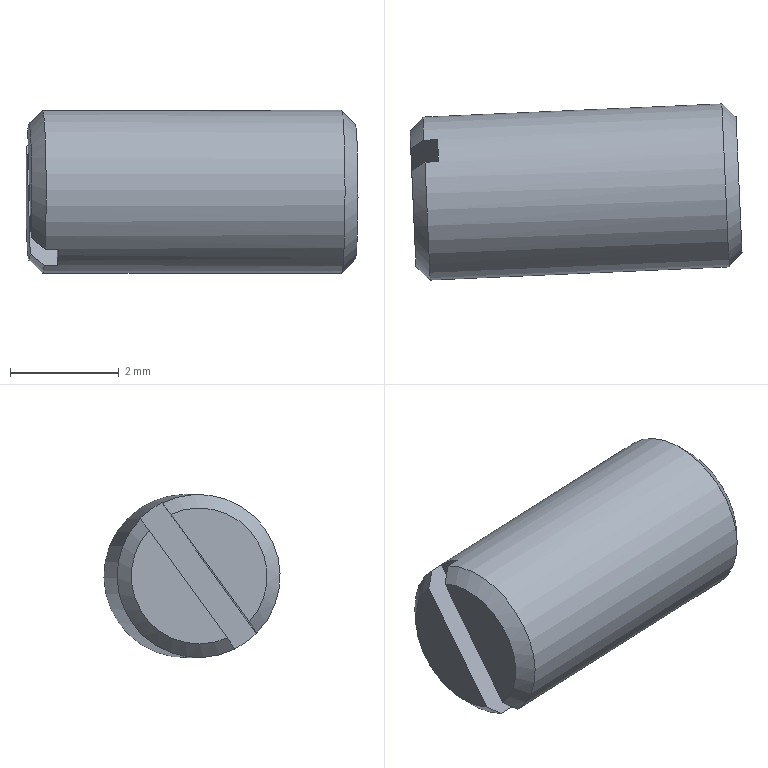Component | NX | SCREW_M3X6 | 1 solid | 10 faces | box 6.1 x 3.24 x 3 mm | volume 41 mm3 | plane 6 | cone 3 | cylinder 1 | commonest cylinder face diameters 3 x1
STEP:
#1=CARTESIAN_POINT('',(0.,0.,0.));
#2=DIRECTION('',(0.,0.,1.));
#3=DIRECTION('',(1.,0.,0.));
#4=AXIS2_PLACEMENT_3D('',#1,#2,#3);
#5=CARTESIAN_POINT('',(-43.719,-0.9021,63.862));
#6=VERTEX_POINT('',#5);
#7=CARTESIAN_POINT('',(-43.782,0.536,65.844));
#8=VERTEX_POINT('',#7);
#9=CARTESIAN_POINT('',(-43.692,-1.51,63.024));
#10=DIRECTION('',(-0.02587,0.5871,0.8091));
#11=VECTOR('',#10,1.);
#12=LINE('',#9,#11);
#13=CARTESIAN_POINT('',(-43.742,-0.3851,65.));
#14=DIRECTION('',(-0.999,-0.04401,0.));
#15=DIRECTION('',(-0.02587,0.5871,0.8091));
#16=AXIS2_PLACEMENT_3D('',#13,#14,#15);
#17=PLANE('',#16);
#18=CARTESIAN_POINT('',(-2.261,0.25));
#19=DIRECTION('',(1.,-0.));
#20=VECTOR('',#19,1.);
#21=LINE('',#18,#20);
#22=(GEOMETRIC_REPRESENTATION_CONTEXT(2)PARAMETRIC_REPRESENTATION_CONTEXT()REPRESENTATION_CONTEXT('',''));
#23=DEFINITIONAL_REPRESENTATION('',(#21),#22);
#24=PCURVE('',#17,#23);
#25=CARTESIAN_POINT('',(-43.192,-1.488,63.024));
#26=DIRECTION('',(0.03561,-0.8083,0.5877));
#27=DIRECTION('',(0.999,0.04401,-0.));
#28=AXIS2_PLACEMENT_3D('',#25,#26,#27);
#29=PLANE('',#28);
#30=CARTESIAN_POINT('',(-0.5,-0.));
#31=DIRECTION('',(0.,1.));
#32=VECTOR('',#31,1.);
#33=LINE('',#30,#32);
#34=(GEOMETRIC_REPRESENTATION_CONTEXT(2)PARAMETRIC_REPRESENTATION_CONTEXT()REPRESENTATION_CONTEXT('',''));
#35=DEFINITIONAL_REPRESENTATION('',(#33),#34);
#36=PCURVE('',#29,#35);
#37=SURFACE_CURVE('',#12,(#24,#36),.PCURVE_S1.);
#38=EDGE_CURVE('',#6,#8,#37,.T.);
#39=ORIENTED_EDGE('',*,*,#38,.T.);
#40=CARTESIAN_POINT('',(-43.742,-0.3851,65.));
#41=DIRECTION('',(-0.999,-0.04401,0.));
#42=DIRECTION('',(-0.02587,0.5871,0.8091));
#43=AXIS2_PLACEMENT_3D('',#40,#41,#42);
#44=CIRCLE('',#43,1.25);
#45=CARTESIAN_POINT('',(0.,0.));
#46=DIRECTION('',(1.,0.));
#47=AXIS2_PLACEMENT_2D('',#45,#46);
#48=CIRCLE('',#47,1.25);
#49=(GEOMETRIC_REPRESENTATION_CONTEXT(2)PARAMETRIC_REPRESENTATION_CONTEXT()REPRESENTATION_CONTEXT('',''));
#50=DEFINITIONAL_REPRESENTATION('',(#48),#49);
#51=PCURVE('',#17,#50);
#52=CARTESIAN_POINT('',(-43.492,-0.3741,65.));
#53=DIRECTION('',(0.999,0.04401,0.));
#54=DIRECTION('',(0.02587,-0.5871,-0.8091));
#55=AXIS2_PLACEMENT_3D('',#52,#53,#54);
#56=CONICAL_SURFACE('',#55,1.5,0.7854);
#57=CARTESIAN_POINT('',(3.142,-0.25));
#58=DIRECTION('',(-1.,0.));
#59=VECTOR('',#58,1.);
#60=LINE('',#57,#59);
#61=(GEOMETRIC_REPRESENTATION_CONTEXT(2)PARAMETRIC_REPRESENTATION_CONTEXT()REPRESENTATION_CONTEXT('',''));
#62=DEFINITIONAL_REPRESENTATION('',(#60),#61);
#63=PCURVE('',#56,#62);
#64=SURFACE_CURVE('',#44,(#51,#63),.PCURVE_S1.);
#65=EDGE_CURVE('',#8,#6,#64,.T.);
#66=ORIENTED_EDGE('',*,*,#65,.T.);
#67=EDGE_LOOP('',(#39,#66));
#68=FACE_BOUND('',#67,.T.);
#69=ADVANCED_FACE('',(#68),#17,.T.);
#70=CARTESIAN_POINT('',(-43.764,0.1318,66.138));
#71=VERTEX_POINT('',#70);
#72=CARTESIAN_POINT('',(-43.701,-1.306,64.156));
#73=VERTEX_POINT('',#72);
#74=CARTESIAN_POINT('',(-43.791,0.7402,66.976));
#75=DIRECTION('',(0.02587,-0.5871,-0.8091));
#76=VECTOR('',#75,1.);
#77=LINE('',#74,#76);
#78=CARTESIAN_POINT('',(-43.742,-0.3851,65.));
#79=DIRECTION('',(-0.999,-0.04401,0.));
#80=DIRECTION('',(-0.02587,0.5871,0.8091));
#81=AXIS2_PLACEMENT_3D('',#78,#79,#80);
#82=PLANE('',#81);
#83=CARTESIAN_POINT('',(2.261,-0.25));
#84=DIRECTION('',(-1.,0.));
#85=VECTOR('',#84,1.);
#86=LINE('',#83,#85);
#87=(GEOMETRIC_REPRESENTATION_CONTEXT(2)PARAMETRIC_REPRESENTATION_CONTEXT()REPRESENTATION_CONTEXT('',''));
#88=DEFINITIONAL_REPRESENTATION('',(#86),#87);
#89=PCURVE('',#82,#88);
#90=CARTESIAN_POINT('',(-43.292,0.7622,66.976));
#91=DIRECTION('',(-0.03561,0.8083,-0.5877));
#92=DIRECTION('',(-0.999,-0.04401,0.));
#93=AXIS2_PLACEMENT_3D('',#90,#91,#92);
#94=PLANE('',#93);
#95=CARTESIAN_POINT('',(0.5,0.));
#96=DIRECTION('',(0.,-1.));
#97=VECTOR('',#96,1.);
#98=LINE('',#95,#97);
#99=(GEOMETRIC_REPRESENTATION_CONTEXT(2)PARAMETRIC_REPRESENTATION_CONTEXT()REPRESENTATION_CONTEXT('',''));
#100=DEFINITIONAL_REPRESENTATION('',(#98),#99);
#101=PCURVE('',#94,#100);
#102=SURFACE_CURVE('',#77,(#89,#101),.PCURVE_S1.);
#103=EDGE_CURVE('',#71,#73,#102,.T.);
#104=ORIENTED_EDGE('',*,*,#103,.T.);
#105=CARTESIAN_POINT('',(-43.742,-0.3851,65.));
#106=DIRECTION('',(-0.999,-0.04401,0.));
#107=DIRECTION('',(-0.02587,0.5871,0.8091));
#108=AXIS2_PLACEMENT_3D('',#105,#106,#107);
#109=CIRCLE('',#108,1.25);
#110=CARTESIAN_POINT('',(0.,0.));
#111=DIRECTION('',(1.,0.));
#112=AXIS2_PLACEMENT_2D('',#110,#111);
#113=CIRCLE('',#112,1.25);
#114=(GEOMETRIC_REPRESENTATION_CONTEXT(2)PARAMETRIC_REPRESENTATION_CONTEXT()REPRESENTATION_CONTEXT('',''));
#115=DEFINITIONAL_REPRESENTATION('',(#113),#114);
#116=PCURVE('',#82,#115);
#117=CARTESIAN_POINT('',(-43.492,-0.3741,65.));
#118=DIRECTION('',(0.999,0.04401,0.));
#119=DIRECTION('',(0.02587,-0.5871,-0.8091));
#120=AXIS2_PLACEMENT_3D('',#117,#118,#119);
#121=CONICAL_SURFACE('',#120,1.5,0.7854);
#122=CARTESIAN_POINT('',(9.425,-0.25));
#123=DIRECTION('',(-1.,0.));
#124=VECTOR('',#123,1.);
#125=LINE('',#122,#124);
#126=(GEOMETRIC_REPRESENTATION_CONTEXT(2)PARAMETRIC_REPRESENTATION_CONTEXT()REPRESENTATION_CONTEXT('',''));
#127=DEFINITIONAL_REPRESENTATION('',(#125),#126);
#128=PCURVE('',#121,#127);
#129=SURFACE_CURVE('',#109,(#116,#128),.PCURVE_S1.);
#130=EDGE_CURVE('',#73,#71,#129,.T.);
#131=ORIENTED_EDGE('',*,*,#130,.T.);
#132=EDGE_LOOP('',(#104,#131));
#133=FACE_BOUND('',#132,.T.);
#134=ADVANCED_FACE('',(#133),#82,.T.);
#135=CARTESIAN_POINT('',(-37.958,-1.013,63.786));
#136=VERTEX_POINT('',#135);
#137=CARTESIAN_POINT('',(-38.044,0.9383,66.05));
#138=VERTEX_POINT('',#137);
#139=CARTESIAN_POINT('',(-37.997,-0.132,65.));
#140=DIRECTION('',(-0.999,-0.04401,0.));
#141=DIRECTION('',(0.02587,-0.5871,-0.8091));
#142=AXIS2_PLACEMENT_3D('',#139,#140,#141);
#143=CIRCLE('',#142,1.5);
#144=CARTESIAN_POINT('',(-37.747,-0.121,65.));
#145=DIRECTION('',(-0.999,-0.04401,0.));
#146=DIRECTION('',(-0.02587,0.5871,0.8091));
#147=AXIS2_PLACEMENT_3D('',#144,#145,#146);
#148=CYLINDRICAL_SURFACE('',#147,1.5);
#149=CARTESIAN_POINT('',(3.142,0.25));
#150=DIRECTION('',(1.,0.));
#151=VECTOR('',#150,1.);
#152=LINE('',#149,#151);
#153=(GEOMETRIC_REPRESENTATION_CONTEXT(2)PARAMETRIC_REPRESENTATION_CONTEXT()REPRESENTATION_CONTEXT('',''));
#154=DEFINITIONAL_REPRESENTATION('',(#152),#153);
#155=PCURVE('',#148,#154);
#156=CARTESIAN_POINT('',(-37.997,-0.132,65.));
#157=DIRECTION('',(-0.999,-0.04401,0.));
#158=DIRECTION('',(-0.02587,0.5871,0.8091));
#159=AXIS2_PLACEMENT_3D('',#156,#157,#158);
#160=CONICAL_SURFACE('',#159,1.5,0.7854);
#161=CARTESIAN_POINT('',(3.142,0.));
#162=DIRECTION('',(1.,0.));
#163=VECTOR('',#162,1.);
#164=LINE('',#161,#163);
#165=(GEOMETRIC_REPRESENTATION_CONTEXT(2)PARAMETRIC_REPRESENTATION_CONTEXT()REPRESENTATION_CONTEXT('',''));
#166=DEFINITIONAL_REPRESENTATION('',(#164),#165);
#167=PCURVE('',#160,#166);
#168=SURFACE_CURVE('',#143,(#155,#167),.PCURVE_S1.);
#169=EDGE_CURVE('',#136,#138,#168,.T.);
#170=ORIENTED_EDGE('',*,*,#169,.T.);
#171=CARTESIAN_POINT('',(-43.289,0.7073,66.05));
#172=VERTEX_POINT('',#171);
#173=CARTESIAN_POINT('',(-38.044,0.9383,66.05));
#174=CARTESIAN_POINT('',(-43.289,0.7073,66.05));
#175=B_SPLINE_CURVE_WITH_KNOTS('',1,(#173,#174),.UNSPECIFIED.,.F.,.F.,(2,2),(0.25,5.5),.PIECEWISE_BEZIER_KNOTS.);
#176=CARTESIAN_POINT('',(6.451,0.));
#177=DIRECTION('',(0.,1.));
#178=VECTOR('',#177,1.);
#179=LINE('',#176,#178);
#180=(GEOMETRIC_REPRESENTATION_CONTEXT(2)PARAMETRIC_REPRESENTATION_CONTEXT()REPRESENTATION_CONTEXT('',''));
#181=DEFINITIONAL_REPRESENTATION('',(#179),#180);
#182=PCURVE('',#148,#181);
#183=CARTESIAN_POINT('',(0.1674,0.));
#184=DIRECTION('',(0.,1.));
#185=VECTOR('',#184,1.);
#186=LINE('',#183,#185);
#187=(GEOMETRIC_REPRESENTATION_CONTEXT(2)PARAMETRIC_REPRESENTATION_CONTEXT()REPRESENTATION_CONTEXT('',''));
#188=DEFINITIONAL_REPRESENTATION('',(#186),#187);
#189=PCURVE('',#148,#188);
#190=SEAM_CURVE('',#175,(#182,#189),.PCURVE_S1.);
#191=EDGE_CURVE('',#138,#172,#190,.T.);
#192=ORIENTED_EDGE('',*,*,#191,.T.);
#193=CARTESIAN_POINT('',(-43.271,0.3031,66.344));
#194=VERTEX_POINT('',#193);
#195=CARTESIAN_POINT('',(-43.242,-0.3631,65.));
#196=DIRECTION('',(-0.999,-0.04401,0.));
#197=DIRECTION('',(0.02587,-0.5871,-0.8091));
#198=AXIS2_PLACEMENT_3D('',#195,#196,#197);
#199=CIRCLE('',#198,1.5);
#200=CARTESIAN_POINT('',(3.142,5.5));
#201=DIRECTION('',(1.,0.));
#202=VECTOR('',#201,1.);
#203=LINE('',#200,#202);
#204=(GEOMETRIC_REPRESENTATION_CONTEXT(2)PARAMETRIC_REPRESENTATION_CONTEXT()REPRESENTATION_CONTEXT('',''));
#205=DEFINITIONAL_REPRESENTATION('',(#203),#204);
#206=PCURVE('',#148,#205);
#207=CARTESIAN_POINT('',(-43.242,-0.3631,65.));
#208=DIRECTION('',(0.999,0.04401,0.));
#209=DIRECTION('',(0.02587,-0.5871,-0.8091));
#210=AXIS2_PLACEMENT_3D('',#207,#208,#209);
#211=PLANE('',#210);
#212=CARTESIAN_POINT('',(1.5,-0.));
#213=CARTESIAN_POINT('',(1.5,-2.598));
#214=CARTESIAN_POINT('',(-0.75,-1.299));
#215=CARTESIAN_POINT('',(-3.,0.));
#216=CARTESIAN_POINT('',(-0.75,1.299));
#217=CARTESIAN_POINT('',(1.5,2.598));
#218=CARTESIAN_POINT('',(1.5,-0.));
#219=(BOUNDED_CURVE()B_SPLINE_CURVE(2,(#212,#213,#214,#215,#216,#217,#218),.UNSPECIFIED.,.T.,.F.)B_SPLINE_CURVE_WITH_KNOTS((1,2,2,2,2,1),(-2.094,0.,2.094,4.189,6.283,8.378),.UNSPECIFIED.)CURVE()GEOMETRIC_REPRESENTATION_ITEM()RATIONAL_B_SPLINE_CURVE((1.,0.5,1.,0.5,1.,0.5,1.))REPRESENTATION_ITEM(''));
#220=(GEOMETRIC_REPRESENTATION_CONTEXT(2)PARAMETRIC_REPRESENTATION_CONTEXT()REPRESENTATION_CONTEXT('',''));
#221=DEFINITIONAL_REPRESENTATION('',(#219),#220);
#222=PCURVE('',#211,#221);
#223=SURFACE_CURVE('',#199,(#206,#222),.PCURVE_S1.);
#224=EDGE_CURVE('',#194,#172,#223,.T.);
#225=ORIENTED_EDGE('',*,*,#224,.F.);
#226=CARTESIAN_POINT('',(-43.521,0.2921,66.344));
#227=VERTEX_POINT('',#226);
#228=CARTESIAN_POINT('',(-37.777,0.5452,66.344));
#229=DIRECTION('',(-0.999,-0.04401,0.));
#230=VECTOR('',#229,1.);
#231=LINE('',#228,#230);
#232=CARTESIAN_POINT('',(6.116,0.));
#233=DIRECTION('',(0.,1.));
#234=VECTOR('',#233,1.);
#235=LINE('',#232,#234);
#236=(GEOMETRIC_REPRESENTATION_CONTEXT(2)PARAMETRIC_REPRESENTATION_CONTEXT()REPRESENTATION_CONTEXT('',''));
#237=DEFINITIONAL_REPRESENTATION('',(#235),#236);
#238=PCURVE('',#148,#237);
#239=CARTESIAN_POINT('',(-5.5,-0.7821));
#240=DIRECTION('',(1.,-0.));
#241=VECTOR('',#240,1.);
#242=LINE('',#239,#241);
#243=(GEOMETRIC_REPRESENTATION_CONTEXT(2)PARAMETRIC_REPRESENTATION_CONTEXT()REPRESENTATION_CONTEXT('',''));
#244=DEFINITIONAL_REPRESENTATION('',(#242),#243);
#245=PCURVE('',#94,#244);
#246=SURFACE_CURVE('',#231,(#238,#245),.PCURVE_S1.);
#247=EDGE_CURVE('',#194,#227,#246,.T.);
#248=ORIENTED_EDGE('',*,*,#247,.T.);
#249=CARTESIAN_POINT('',(-43.445,-1.445,63.95));
#250=VERTEX_POINT('',#249);
#251=CARTESIAN_POINT('',(-43.492,-0.3741,65.));
#252=DIRECTION('',(0.999,0.04401,-0.));
#253=DIRECTION('',(-0.02587,0.5871,0.8091));
#254=AXIS2_PLACEMENT_3D('',#251,#252,#253);
#255=CIRCLE('',#254,1.5);
#256=CARTESIAN_POINT('',(6.283,5.75));
#257=DIRECTION('',(-1.,0.));
#258=VECTOR('',#257,1.);
#259=LINE('',#256,#258);
#260=(GEOMETRIC_REPRESENTATION_CONTEXT(2)PARAMETRIC_REPRESENTATION_CONTEXT()REPRESENTATION_CONTEXT('',''));
#261=DEFINITIONAL_REPRESENTATION('',(#259),#260);
#262=PCURVE('',#148,#261);
#263=CARTESIAN_POINT('',(3.142,0.));
#264=DIRECTION('',(1.,-0.));
#265=VECTOR('',#264,1.);
#266=LINE('',#263,#265);
#267=(GEOMETRIC_REPRESENTATION_CONTEXT(2)PARAMETRIC_REPRESENTATION_CONTEXT()REPRESENTATION_CONTEXT('',''));
#268=DEFINITIONAL_REPRESENTATION('',(#266),#267);
#269=PCURVE('',#121,#268);
#270=SURFACE_CURVE('',#255,(#262,#269),.PCURVE_S1.);
#271=EDGE_CURVE('',#227,#250,#270,.T.);
#272=ORIENTED_EDGE('',*,*,#271,.T.);
#273=CARTESIAN_POINT('',(-43.195,-1.434,63.95));
#274=VERTEX_POINT('',#273);
#275=CARTESIAN_POINT('',(-37.7,-1.191,63.95));
#276=DIRECTION('',(0.999,0.04401,0.));
#277=VECTOR('',#276,1.);
#278=LINE('',#275,#277);
#279=CARTESIAN_POINT('',(3.309,-0.));
#280=DIRECTION('',(0.,-1.));
#281=VECTOR('',#280,1.);
#282=LINE('',#279,#281);
#283=(GEOMETRIC_REPRESENTATION_CONTEXT(2)PARAMETRIC_REPRESENTATION_CONTEXT()REPRESENTATION_CONTEXT('',''));
#284=DEFINITIONAL_REPRESENTATION('',(#282),#283);
#285=PCURVE('',#148,#284);
#286=CARTESIAN_POINT('',(-5.5,-3.74));
#287=DIRECTION('',(-1.,0.));
#288=VECTOR('',#287,1.);
#289=LINE('',#286,#288);
#290=(GEOMETRIC_REPRESENTATION_CONTEXT(2)PARAMETRIC_REPRESENTATION_CONTEXT()REPRESENTATION_CONTEXT('',''));
#291=DEFINITIONAL_REPRESENTATION('',(#289),#290);
#292=PCURVE('',#94,#291);
#293=SURFACE_CURVE('',#278,(#285,#292),.PCURVE_S1.);
#294=EDGE_CURVE('',#250,#274,#293,.T.);
#295=ORIENTED_EDGE('',*,*,#294,.T.);
#296=CARTESIAN_POINT('',(-43.213,-1.029,63.656));
#297=VERTEX_POINT('',#296);
#298=CARTESIAN_POINT('',(-43.242,-0.3631,65.));
#299=DIRECTION('',(-0.999,-0.04401,0.));
#300=DIRECTION('',(0.02587,-0.5871,-0.8091));
#301=AXIS2_PLACEMENT_3D('',#298,#299,#300);
#302=CIRCLE('',#301,1.5);
#303=CARTESIAN_POINT('',(-3.142,5.5));
#304=DIRECTION('',(1.,-0.));
#305=VECTOR('',#304,1.);
#306=LINE('',#303,#305);
#307=(GEOMETRIC_REPRESENTATION_CONTEXT(2)PARAMETRIC_REPRESENTATION_CONTEXT()REPRESENTATION_CONTEXT('',''));
#308=DEFINITIONAL_REPRESENTATION('',(#306),#307);
#309=PCURVE('',#148,#308);
#310=CARTESIAN_POINT('',(1.5,-0.));
#311=CARTESIAN_POINT('',(1.5,-2.598));
#312=CARTESIAN_POINT('',(-0.75,-1.299));
#313=CARTESIAN_POINT('',(-3.,0.));
#314=CARTESIAN_POINT('',(-0.75,1.299));
#315=CARTESIAN_POINT('',(1.5,2.598));
#316=CARTESIAN_POINT('',(1.5,-0.));
#317=(BOUNDED_CURVE()B_SPLINE_CURVE(2,(#310,#311,#312,#313,#314,#315,#316),.UNSPECIFIED.,.T.,.F.)B_SPLINE_CURVE_WITH_KNOTS((1,2,2,2,2,1),(-2.094,0.,2.094,4.189,6.283,8.378),.UNSPECIFIED.)CURVE()GEOMETRIC_REPRESENTATION_ITEM()RATIONAL_B_SPLINE_CURVE((1.,0.5,1.,0.5,1.,0.5,1.))REPRESENTATION_ITEM(''));
#318=(GEOMETRIC_REPRESENTATION_CONTEXT(2)PARAMETRIC_REPRESENTATION_CONTEXT()REPRESENTATION_CONTEXT('',''));
#319=DEFINITIONAL_REPRESENTATION('',(#317),#318);
#320=PCURVE('',#211,#319);
#321=SURFACE_CURVE('',#302,(#309,#320),.PCURVE_S1.);
#322=EDGE_CURVE('',#297,#274,#321,.T.);
#323=ORIENTED_EDGE('',*,*,#322,.F.);
#324=CARTESIAN_POINT('',(-43.462,-1.04,63.656));
#325=VERTEX_POINT('',#324);
#326=CARTESIAN_POINT('',(-37.718,-0.7873,63.656));
#327=DIRECTION('',(-0.999,-0.04401,0.));
#328=VECTOR('',#327,1.);
#329=LINE('',#326,#328);
#330=CARTESIAN_POINT('',(2.974,-0.));
#331=DIRECTION('',(0.,1.));
#332=VECTOR('',#331,1.);
#333=LINE('',#330,#332);
#334=(GEOMETRIC_REPRESENTATION_CONTEXT(2)PARAMETRIC_REPRESENTATION_CONTEXT()REPRESENTATION_CONTEXT('',''));
#335=DEFINITIONAL_REPRESENTATION('',(#333),#334);
#336=PCURVE('',#148,#335);
#337=CARTESIAN_POINT('',(5.5,0.7821));
#338=DIRECTION('',(-1.,-0.));
#339=VECTOR('',#338,1.);
#340=LINE('',#337,#339);
#341=(GEOMETRIC_REPRESENTATION_CONTEXT(2)PARAMETRIC_REPRESENTATION_CONTEXT()REPRESENTATION_CONTEXT('',''));
#342=DEFINITIONAL_REPRESENTATION('',(#340),#341);
#343=PCURVE('',#29,#342);
#344=SURFACE_CURVE('',#329,(#336,#343),.PCURVE_S1.);
#345=EDGE_CURVE('',#297,#325,#344,.T.);
#346=ORIENTED_EDGE('',*,*,#345,.T.);
#347=CARTESIAN_POINT('',(-43.539,0.6963,66.05));
#348=VERTEX_POINT('',#347);
#349=CARTESIAN_POINT('',(-43.492,-0.3741,65.));
#350=DIRECTION('',(0.999,0.04401,-0.));
#351=DIRECTION('',(-0.02587,0.5871,0.8091));
#352=AXIS2_PLACEMENT_3D('',#349,#350,#351);
#353=CIRCLE('',#352,1.5);
#354=CARTESIAN_POINT('',(6.283,5.75));
#355=DIRECTION('',(-1.,0.));
#356=VECTOR('',#355,1.);
#357=LINE('',#354,#356);
#358=(GEOMETRIC_REPRESENTATION_CONTEXT(2)PARAMETRIC_REPRESENTATION_CONTEXT()REPRESENTATION_CONTEXT('',''));
#359=DEFINITIONAL_REPRESENTATION('',(#357),#358);
#360=PCURVE('',#148,#359);
#361=CARTESIAN_POINT('',(-3.142,0.));
#362=DIRECTION('',(1.,-0.));
#363=VECTOR('',#362,1.);
#364=LINE('',#361,#363);
#365=(GEOMETRIC_REPRESENTATION_CONTEXT(2)PARAMETRIC_REPRESENTATION_CONTEXT()REPRESENTATION_CONTEXT('',''));
#366=DEFINITIONAL_REPRESENTATION('',(#364),#365);
#367=PCURVE('',#56,#366);
#368=SURFACE_CURVE('',#353,(#360,#367),.PCURVE_S1.);
#369=EDGE_CURVE('',#325,#348,#368,.T.);
#370=ORIENTED_EDGE('',*,*,#369,.T.);
#371=CARTESIAN_POINT('',(-37.794,0.9493,66.05));
#372=DIRECTION('',(0.999,0.04401,0.));
#373=VECTOR('',#372,1.);
#374=LINE('',#371,#373);
#375=CARTESIAN_POINT('',(0.1674,-0.));
#376=DIRECTION('',(0.,-1.));
#377=VECTOR('',#376,1.);
#378=LINE('',#375,#377);
#379=(GEOMETRIC_REPRESENTATION_CONTEXT(2)PARAMETRIC_REPRESENTATION_CONTEXT()REPRESENTATION_CONTEXT('',''));
#380=DEFINITIONAL_REPRESENTATION('',(#378),#379);
#381=PCURVE('',#148,#380);
#382=CARTESIAN_POINT('',(5.5,3.74));
#383=DIRECTION('',(1.,0.));
#384=VECTOR('',#383,1.);
#385=LINE('',#382,#384);
#386=(GEOMETRIC_REPRESENTATION_CONTEXT(2)PARAMETRIC_REPRESENTATION_CONTEXT()REPRESENTATION_CONTEXT('',''));
#387=DEFINITIONAL_REPRESENTATION('',(#385),#386);
#388=PCURVE('',#29,#387);
#389=SURFACE_CURVE('',#374,(#381,#388),.PCURVE_S1.);
#390=EDGE_CURVE('',#348,#172,#389,.T.);
#391=ORIENTED_EDGE('',*,*,#390,.T.);
#392=ORIENTED_EDGE('',*,*,#191,.F.);
#393=CARTESIAN_POINT('',(-37.997,-0.132,65.));
#394=DIRECTION('',(-0.999,-0.04401,0.));
#395=DIRECTION('',(0.02587,-0.5871,-0.8091));
#396=AXIS2_PLACEMENT_3D('',#393,#394,#395);
#397=CIRCLE('',#396,1.5);
#398=CARTESIAN_POINT('',(-3.142,0.25));
#399=DIRECTION('',(1.,0.));
#400=VECTOR('',#399,1.);
#401=LINE('',#398,#400);
#402=(GEOMETRIC_REPRESENTATION_CONTEXT(2)PARAMETRIC_REPRESENTATION_CONTEXT()REPRESENTATION_CONTEXT('',''));
#403=DEFINITIONAL_REPRESENTATION('',(#401),#402);
#404=PCURVE('',#148,#403);
#405=CARTESIAN_POINT('',(3.142,0.));
#406=DIRECTION('',(1.,-0.));
#407=VECTOR('',#406,1.);
#408=LINE('',#405,#407);
#409=(GEOMETRIC_REPRESENTATION_CONTEXT(2)PARAMETRIC_REPRESENTATION_CONTEXT()REPRESENTATION_CONTEXT('',''));
#410=DEFINITIONAL_REPRESENTATION('',(#408),#409);
#411=PCURVE('',#160,#410);
#412=SURFACE_CURVE('',#397,(#404,#411),.PCURVE_S1.);
#413=EDGE_CURVE('',#138,#136,#412,.T.);
#414=ORIENTED_EDGE('',*,*,#413,.T.);
#415=EDGE_LOOP('',(#170,#192,#225,#248,#272,#295,#323,#346,#370,#391,#392,#414));
#416=FACE_BOUND('',#415,.T.);
#417=ADVANCED_FACE('',(#416),#148,.T.);
#418=CARTESIAN_POINT('',(-37.715,-0.8549,63.989));
#419=VERTEX_POINT('',#418);
#420=CARTESIAN_POINT('',(-37.747,-0.121,65.));
#421=DIRECTION('',(0.999,0.04401,0.));
#422=DIRECTION('',(0.02587,-0.5871,-0.8091));
#423=AXIS2_PLACEMENT_3D('',#420,#421,#422);
#424=CIRCLE('',#423,1.25);
#425=CARTESIAN_POINT('',(-37.747,-0.121,65.));
#426=DIRECTION('',(0.999,0.04401,0.));
#427=DIRECTION('',(0.02587,-0.5871,-0.8091));
#428=AXIS2_PLACEMENT_3D('',#425,#426,#427);
#429=PLANE('',#428);
#430=CARTESIAN_POINT('',(0.,0.));
#431=DIRECTION('',(1.,-0.));
#432=AXIS2_PLACEMENT_2D('',#430,#431);
#433=CIRCLE('',#432,1.25);
#434=(GEOMETRIC_REPRESENTATION_CONTEXT(2)PARAMETRIC_REPRESENTATION_CONTEXT()REPRESENTATION_CONTEXT('',''));
#435=DEFINITIONAL_REPRESENTATION('',(#433),#434);
#436=PCURVE('',#429,#435);
#437=CARTESIAN_POINT('',(9.425,-0.25));
#438=DIRECTION('',(-1.,0.));
#439=VECTOR('',#438,1.);
#440=LINE('',#437,#439);
#441=(GEOMETRIC_REPRESENTATION_CONTEXT(2)PARAMETRIC_REPRESENTATION_CONTEXT()REPRESENTATION_CONTEXT('',''));
#442=DEFINITIONAL_REPRESENTATION('',(#440),#441);
#443=PCURVE('',#160,#442);
#444=SURFACE_CURVE('',#424,(#436,#443),.PCURVE_S1.);
#445=EDGE_CURVE('',#419,#419,#444,.T.);
#446=ORIENTED_EDGE('',*,*,#445,.T.);
#447=EDGE_LOOP('',(#446));
#448=FACE_BOUND('',#447,.T.);
#449=ADVANCED_FACE('',(#448),#429,.T.);
#450=ORIENTED_EDGE('',*,*,#445,.F.);
#451=CARTESIAN_POINT('',(-37.715,-0.8549,63.989));
#452=CARTESIAN_POINT('',(-37.958,-1.013,63.786));
#453=B_SPLINE_CURVE_WITH_KNOTS('',1,(#451,#452),.UNSPECIFIED.,.F.,.F.,(2,2),(-0.3536,0.),.PIECEWISE_BEZIER_KNOTS.);
#454=CARTESIAN_POINT('',(9.425,0.));
#455=DIRECTION('',(0.,1.));
#456=VECTOR('',#455,1.);
#457=LINE('',#454,#456);
#458=(GEOMETRIC_REPRESENTATION_CONTEXT(2)PARAMETRIC_REPRESENTATION_CONTEXT()REPRESENTATION_CONTEXT('',''));
#459=DEFINITIONAL_REPRESENTATION('',(#457),#458);
#460=PCURVE('',#160,#459);
#461=CARTESIAN_POINT('',(3.142,0.));
#462=DIRECTION('',(0.,1.));
#463=VECTOR('',#462,1.);
#464=LINE('',#461,#463);
#465=(GEOMETRIC_REPRESENTATION_CONTEXT(2)PARAMETRIC_REPRESENTATION_CONTEXT()REPRESENTATION_CONTEXT('',''));
#466=DEFINITIONAL_REPRESENTATION('',(#464),#465);
#467=PCURVE('',#160,#466);
#468=SEAM_CURVE('',#453,(#460,#467),.PCURVE_S1.);
#469=EDGE_CURVE('',#419,#136,#468,.T.);
#470=ORIENTED_EDGE('',*,*,#469,.T.);
#471=ORIENTED_EDGE('',*,*,#413,.F.);
#472=ORIENTED_EDGE('',*,*,#169,.F.);
#473=ORIENTED_EDGE('',*,*,#469,.F.);
#474=EDGE_LOOP('',(#450,#470,#471,#472,#473));
#475=FACE_BOUND('',#474,.T.);
#476=ADVANCED_FACE('',(#475),#160,.T.);
#477=ORIENTED_EDGE('',*,*,#294,.F.);
#478=CARTESIAN_POINT('',(-43.445,-1.445,63.95));
#479=CARTESIAN_POINT('',(-43.53,-1.398,64.019));
#480=CARTESIAN_POINT('',(-43.616,-1.352,64.087));
#481=CARTESIAN_POINT('',(-43.701,-1.306,64.156));
#482=B_SPLINE_CURVE_WITH_KNOTS('',3,(#478,#479,#480,#481),.UNSPECIFIED.,.F.,.F.,(4,4),(0.,1.),.PIECEWISE_BEZIER_KNOTS.);
#483=CARTESIAN_POINT('',(0.25,-3.74));
#484=CARTESIAN_POINT('',(0.3335,-3.655));
#485=CARTESIAN_POINT('',(0.4168,-3.571));
#486=CARTESIAN_POINT('',(0.5,-3.486));
#487=B_SPLINE_CURVE_WITH_KNOTS('',3,(#483,#484,#485,#486),.UNSPECIFIED.,.F.,.F.,(4,4),(0.,1.),.PIECEWISE_BEZIER_KNOTS.);
#488=(GEOMETRIC_REPRESENTATION_CONTEXT(2)PARAMETRIC_REPRESENTATION_CONTEXT()REPRESENTATION_CONTEXT('',''));
#489=DEFINITIONAL_REPRESENTATION('',(#487),#488);
#490=PCURVE('',#94,#489);
#491=CARTESIAN_POINT('',(6.116,-0.));
#492=CARTESIAN_POINT('',(6.082,-0.25));
#493=B_SPLINE_CURVE_WITH_KNOTS('',1,(#491,#492),.UNSPECIFIED.,.F.,.F.,(2,2),(0.,1.),.PIECEWISE_BEZIER_KNOTS.);
#494=(GEOMETRIC_REPRESENTATION_CONTEXT(2)PARAMETRIC_REPRESENTATION_CONTEXT()REPRESENTATION_CONTEXT('',''));
#495=DEFINITIONAL_REPRESENTATION('',(#493),#494);
#496=PCURVE('',#121,#495);
#497=SURFACE_CURVE('',#482,(#490,#496),.PCURVE_S1.);
#498=EDGE_CURVE('',#250,#73,#497,.T.);
#499=ORIENTED_EDGE('',*,*,#498,.T.);
#500=ORIENTED_EDGE('',*,*,#103,.F.);
#501=CARTESIAN_POINT('',(-43.764,0.1318,66.138));
#502=CARTESIAN_POINT('',(-43.683,0.1853,66.207));
#503=CARTESIAN_POINT('',(-43.602,0.2387,66.275));
#504=CARTESIAN_POINT('',(-43.521,0.2921,66.344));
#505=B_SPLINE_CURVE_WITH_KNOTS('',3,(#501,#502,#503,#504),.UNSPECIFIED.,.F.,.F.,(4,4),(0.,1.),.PIECEWISE_BEZIER_KNOTS.);
#506=CARTESIAN_POINT('',(0.5,-1.036));
#507=CARTESIAN_POINT('',(0.4168,-0.9514));
#508=CARTESIAN_POINT('',(0.3335,-0.8667));
#509=CARTESIAN_POINT('',(0.25,-0.7821));
#510=B_SPLINE_CURVE_WITH_KNOTS('',3,(#506,#507,#508,#509),.UNSPECIFIED.,.F.,.F.,(4,4),(0.,1.),.PIECEWISE_BEZIER_KNOTS.);
#511=(GEOMETRIC_REPRESENTATION_CONTEXT(2)PARAMETRIC_REPRESENTATION_CONTEXT()REPRESENTATION_CONTEXT('',''));
#512=DEFINITIONAL_REPRESENTATION('',(#510),#511);
#513=PCURVE('',#94,#512);
#514=CARTESIAN_POINT('',(3.343,-0.25));
#515=CARTESIAN_POINT('',(3.309,-0.));
#516=B_SPLINE_CURVE_WITH_KNOTS('',1,(#514,#515),.UNSPECIFIED.,.F.,.F.,(2,2),(0.,1.),.PIECEWISE_BEZIER_KNOTS.);
#517=(GEOMETRIC_REPRESENTATION_CONTEXT(2)PARAMETRIC_REPRESENTATION_CONTEXT()REPRESENTATION_CONTEXT('',''));
#518=DEFINITIONAL_REPRESENTATION('',(#516),#517);
#519=PCURVE('',#121,#518);
#520=SURFACE_CURVE('',#505,(#513,#519),.PCURVE_S1.);
#521=EDGE_CURVE('',#71,#227,#520,.T.);
#522=ORIENTED_EDGE('',*,*,#521,.T.);
#523=ORIENTED_EDGE('',*,*,#247,.F.);
#524=CARTESIAN_POINT('',(-43.292,0.7622,66.976));
#525=DIRECTION('',(-0.02587,0.5871,0.8091));
#526=VECTOR('',#525,1.);
#527=LINE('',#524,#526);
#528=CARTESIAN_POINT('',(0.,0.));
#529=DIRECTION('',(-0.,1.));
#530=VECTOR('',#529,1.);
#531=LINE('',#528,#530);
#532=(GEOMETRIC_REPRESENTATION_CONTEXT(2)PARAMETRIC_REPRESENTATION_CONTEXT()REPRESENTATION_CONTEXT('',''));
#533=DEFINITIONAL_REPRESENTATION('',(#531),#532);
#534=PCURVE('',#94,#533);
#535=CARTESIAN_POINT('',(-2.261,-0.25));
#536=DIRECTION('',(-1.,-0.));
#537=VECTOR('',#536,1.);
#538=LINE('',#535,#537);
#539=(GEOMETRIC_REPRESENTATION_CONTEXT(2)PARAMETRIC_REPRESENTATION_CONTEXT()REPRESENTATION_CONTEXT('',''));
#540=DEFINITIONAL_REPRESENTATION('',(#538),#539);
#541=PCURVE('',#211,#540);
#542=SURFACE_CURVE('',#527,(#534,#541),.PCURVE_S1.);
#543=EDGE_CURVE('',#274,#194,#542,.T.);
#544=ORIENTED_EDGE('',*,*,#543,.F.);
#545=EDGE_LOOP('',(#477,#499,#500,#522,#523,#544));
#546=FACE_BOUND('',#545,.T.);
#547=ADVANCED_FACE('',(#546),#94,.T.);
#548=ORIENTED_EDGE('',*,*,#390,.F.);
#549=CARTESIAN_POINT('',(-43.539,0.6963,66.05));
#550=CARTESIAN_POINT('',(-43.62,0.6429,65.981));
#551=CARTESIAN_POINT('',(-43.701,0.5895,65.913));
#552=CARTESIAN_POINT('',(-43.782,0.536,65.844));
#553=B_SPLINE_CURVE_WITH_KNOTS('',3,(#549,#550,#551,#552),.UNSPECIFIED.,.F.,.F.,(4,4),(0.,1.),.PIECEWISE_BEZIER_KNOTS.);
#554=CARTESIAN_POINT('',(-0.25,3.74));
#555=CARTESIAN_POINT('',(-0.3335,3.655));
#556=CARTESIAN_POINT('',(-0.4168,3.571));
#557=CARTESIAN_POINT('',(-0.5,3.486));
#558=B_SPLINE_CURVE_WITH_KNOTS('',3,(#554,#555,#556,#557),.UNSPECIFIED.,.F.,.F.,(4,4),(0.,1.),.PIECEWISE_BEZIER_KNOTS.);
#559=(GEOMETRIC_REPRESENTATION_CONTEXT(2)PARAMETRIC_REPRESENTATION_CONTEXT()REPRESENTATION_CONTEXT('',''));
#560=DEFINITIONAL_REPRESENTATION('',(#558),#559);
#561=PCURVE('',#29,#560);
#562=CARTESIAN_POINT('',(2.974,-0.));
#563=CARTESIAN_POINT('',(2.94,-0.25));
#564=B_SPLINE_CURVE_WITH_KNOTS('',1,(#562,#563),.UNSPECIFIED.,.F.,.F.,(2,2),(0.,1.),.PIECEWISE_BEZIER_KNOTS.);
#565=(GEOMETRIC_REPRESENTATION_CONTEXT(2)PARAMETRIC_REPRESENTATION_CONTEXT()REPRESENTATION_CONTEXT('',''));
#566=DEFINITIONAL_REPRESENTATION('',(#564),#565);
#567=PCURVE('',#56,#566);
#568=SURFACE_CURVE('',#553,(#561,#567),.PCURVE_S1.);
#569=EDGE_CURVE('',#348,#8,#568,.T.);
#570=ORIENTED_EDGE('',*,*,#569,.T.);
#571=ORIENTED_EDGE('',*,*,#38,.F.);
#572=CARTESIAN_POINT('',(-43.719,-0.9021,63.862));
#573=CARTESIAN_POINT('',(-43.633,-0.9483,63.793));
#574=CARTESIAN_POINT('',(-43.548,-0.9943,63.725));
#575=CARTESIAN_POINT('',(-43.462,-1.04,63.656));
#576=B_SPLINE_CURVE_WITH_KNOTS('',3,(#572,#573,#574,#575),.UNSPECIFIED.,.F.,.F.,(4,4),(0.,1.),.PIECEWISE_BEZIER_KNOTS.);
#577=CARTESIAN_POINT('',(-0.5,1.036));
#578=CARTESIAN_POINT('',(-0.4168,0.9514));
#579=CARTESIAN_POINT('',(-0.3335,0.8667));
#580=CARTESIAN_POINT('',(-0.25,0.7821));
#581=B_SPLINE_CURVE_WITH_KNOTS('',3,(#577,#578,#579,#580),.UNSPECIFIED.,.F.,.F.,(4,4),(0.,1.),.PIECEWISE_BEZIER_KNOTS.);
#582=(GEOMETRIC_REPRESENTATION_CONTEXT(2)PARAMETRIC_REPRESENTATION_CONTEXT()REPRESENTATION_CONTEXT('',''));
#583=DEFINITIONAL_REPRESENTATION('',(#581),#582);
#584=PCURVE('',#29,#583);
#585=CARTESIAN_POINT('',(0.2014,-0.25));
#586=CARTESIAN_POINT('',(0.1674,0.));
#587=B_SPLINE_CURVE_WITH_KNOTS('',1,(#585,#586),.UNSPECIFIED.,.F.,.F.,(2,2),(0.,1.),.PIECEWISE_BEZIER_KNOTS.);
#588=(GEOMETRIC_REPRESENTATION_CONTEXT(2)PARAMETRIC_REPRESENTATION_CONTEXT()REPRESENTATION_CONTEXT('',''));
#589=DEFINITIONAL_REPRESENTATION('',(#587),#588);
#590=PCURVE('',#56,#589);
#591=SURFACE_CURVE('',#576,(#584,#590),.PCURVE_S1.);
#592=EDGE_CURVE('',#6,#325,#591,.T.);
#593=ORIENTED_EDGE('',*,*,#592,.T.);
#594=ORIENTED_EDGE('',*,*,#345,.F.);
#595=CARTESIAN_POINT('',(-43.192,-1.488,63.024));
#596=DIRECTION('',(0.02587,-0.5871,-0.8091));
#597=VECTOR('',#596,1.);
#598=LINE('',#595,#597);
#599=CARTESIAN_POINT('',(0.,0.));
#600=DIRECTION('',(-0.,-1.));
#601=VECTOR('',#600,1.);
#602=LINE('',#599,#601);
#603=(GEOMETRIC_REPRESENTATION_CONTEXT(2)PARAMETRIC_REPRESENTATION_CONTEXT()REPRESENTATION_CONTEXT('',''));
#604=DEFINITIONAL_REPRESENTATION('',(#602),#603);
#605=PCURVE('',#29,#604);
#606=CARTESIAN_POINT('',(2.261,0.25));
#607=DIRECTION('',(1.,0.));
#608=VECTOR('',#607,1.);
#609=LINE('',#606,#608);
#610=(GEOMETRIC_REPRESENTATION_CONTEXT(2)PARAMETRIC_REPRESENTATION_CONTEXT()REPRESENTATION_CONTEXT('',''));
#611=DEFINITIONAL_REPRESENTATION('',(#609),#610);
#612=PCURVE('',#211,#611);
#613=SURFACE_CURVE('',#598,(#605,#612),.PCURVE_S1.);
#614=EDGE_CURVE('',#172,#297,#613,.T.);
#615=ORIENTED_EDGE('',*,*,#614,.F.);
#616=EDGE_LOOP('',(#548,#570,#571,#593,#594,#615));
#617=FACE_BOUND('',#616,.T.);
#618=ADVANCED_FACE('',(#617),#29,.T.);
#619=ORIENTED_EDGE('',*,*,#224,.T.);
#620=ORIENTED_EDGE('',*,*,#614,.T.);
#621=ORIENTED_EDGE('',*,*,#322,.T.);
#622=ORIENTED_EDGE('',*,*,#543,.T.);
#623=EDGE_LOOP('',(#619,#620,#621,#622));
#624=FACE_BOUND('',#623,.T.);
#625=ADVANCED_FACE('',(#624),#211,.F.);
#626=ORIENTED_EDGE('',*,*,#592,.F.);
#627=ORIENTED_EDGE('',*,*,#65,.F.);
#628=ORIENTED_EDGE('',*,*,#569,.F.);
#629=ORIENTED_EDGE('',*,*,#369,.F.);
#630=EDGE_LOOP('',(#626,#627,#628,#629));
#631=FACE_BOUND('',#630,.T.);
#632=ADVANCED_FACE('',(#631),#56,.T.);
#633=ORIENTED_EDGE('',*,*,#521,.F.);
#634=ORIENTED_EDGE('',*,*,#130,.F.);
#635=ORIENTED_EDGE('',*,*,#498,.F.);
#636=ORIENTED_EDGE('',*,*,#271,.F.);
#637=EDGE_LOOP('',(#633,#634,#635,#636));
#638=FACE_BOUND('',#637,.T.);
#639=ADVANCED_FACE('',(#638),#121,.T.);
#640=CLOSED_SHELL('',(#69,#134,#417,#449,#476,#547,#618,#625,#632,#639));
#641=MANIFOLD_SOLID_BREP('',#640);
#642=(LENGTH_UNIT()NAMED_UNIT(*)SI_UNIT(.MILLI.,.METRE.));
#643=UNCERTAINTY_MEASURE_WITH_UNIT(LENGTH_MEASURE(0.001),#642,'','');
#644=(NAMED_UNIT(*)PLANE_ANGLE_UNIT()SI_UNIT($,.RADIAN.));
#645=(NAMED_UNIT(*)SI_UNIT($,.STERADIAN.)SOLID_ANGLE_UNIT());
#646=(GEOMETRIC_REPRESENTATION_CONTEXT(3)GLOBAL_UNCERTAINTY_ASSIGNED_CONTEXT((#643))GLOBAL_UNIT_ASSIGNED_CONTEXT((#642,#644,#645))REPRESENTATION_CONTEXT('',''));
#647=ADVANCED_BREP_SHAPE_REPRESENTATION('',(#4,#641),#646);